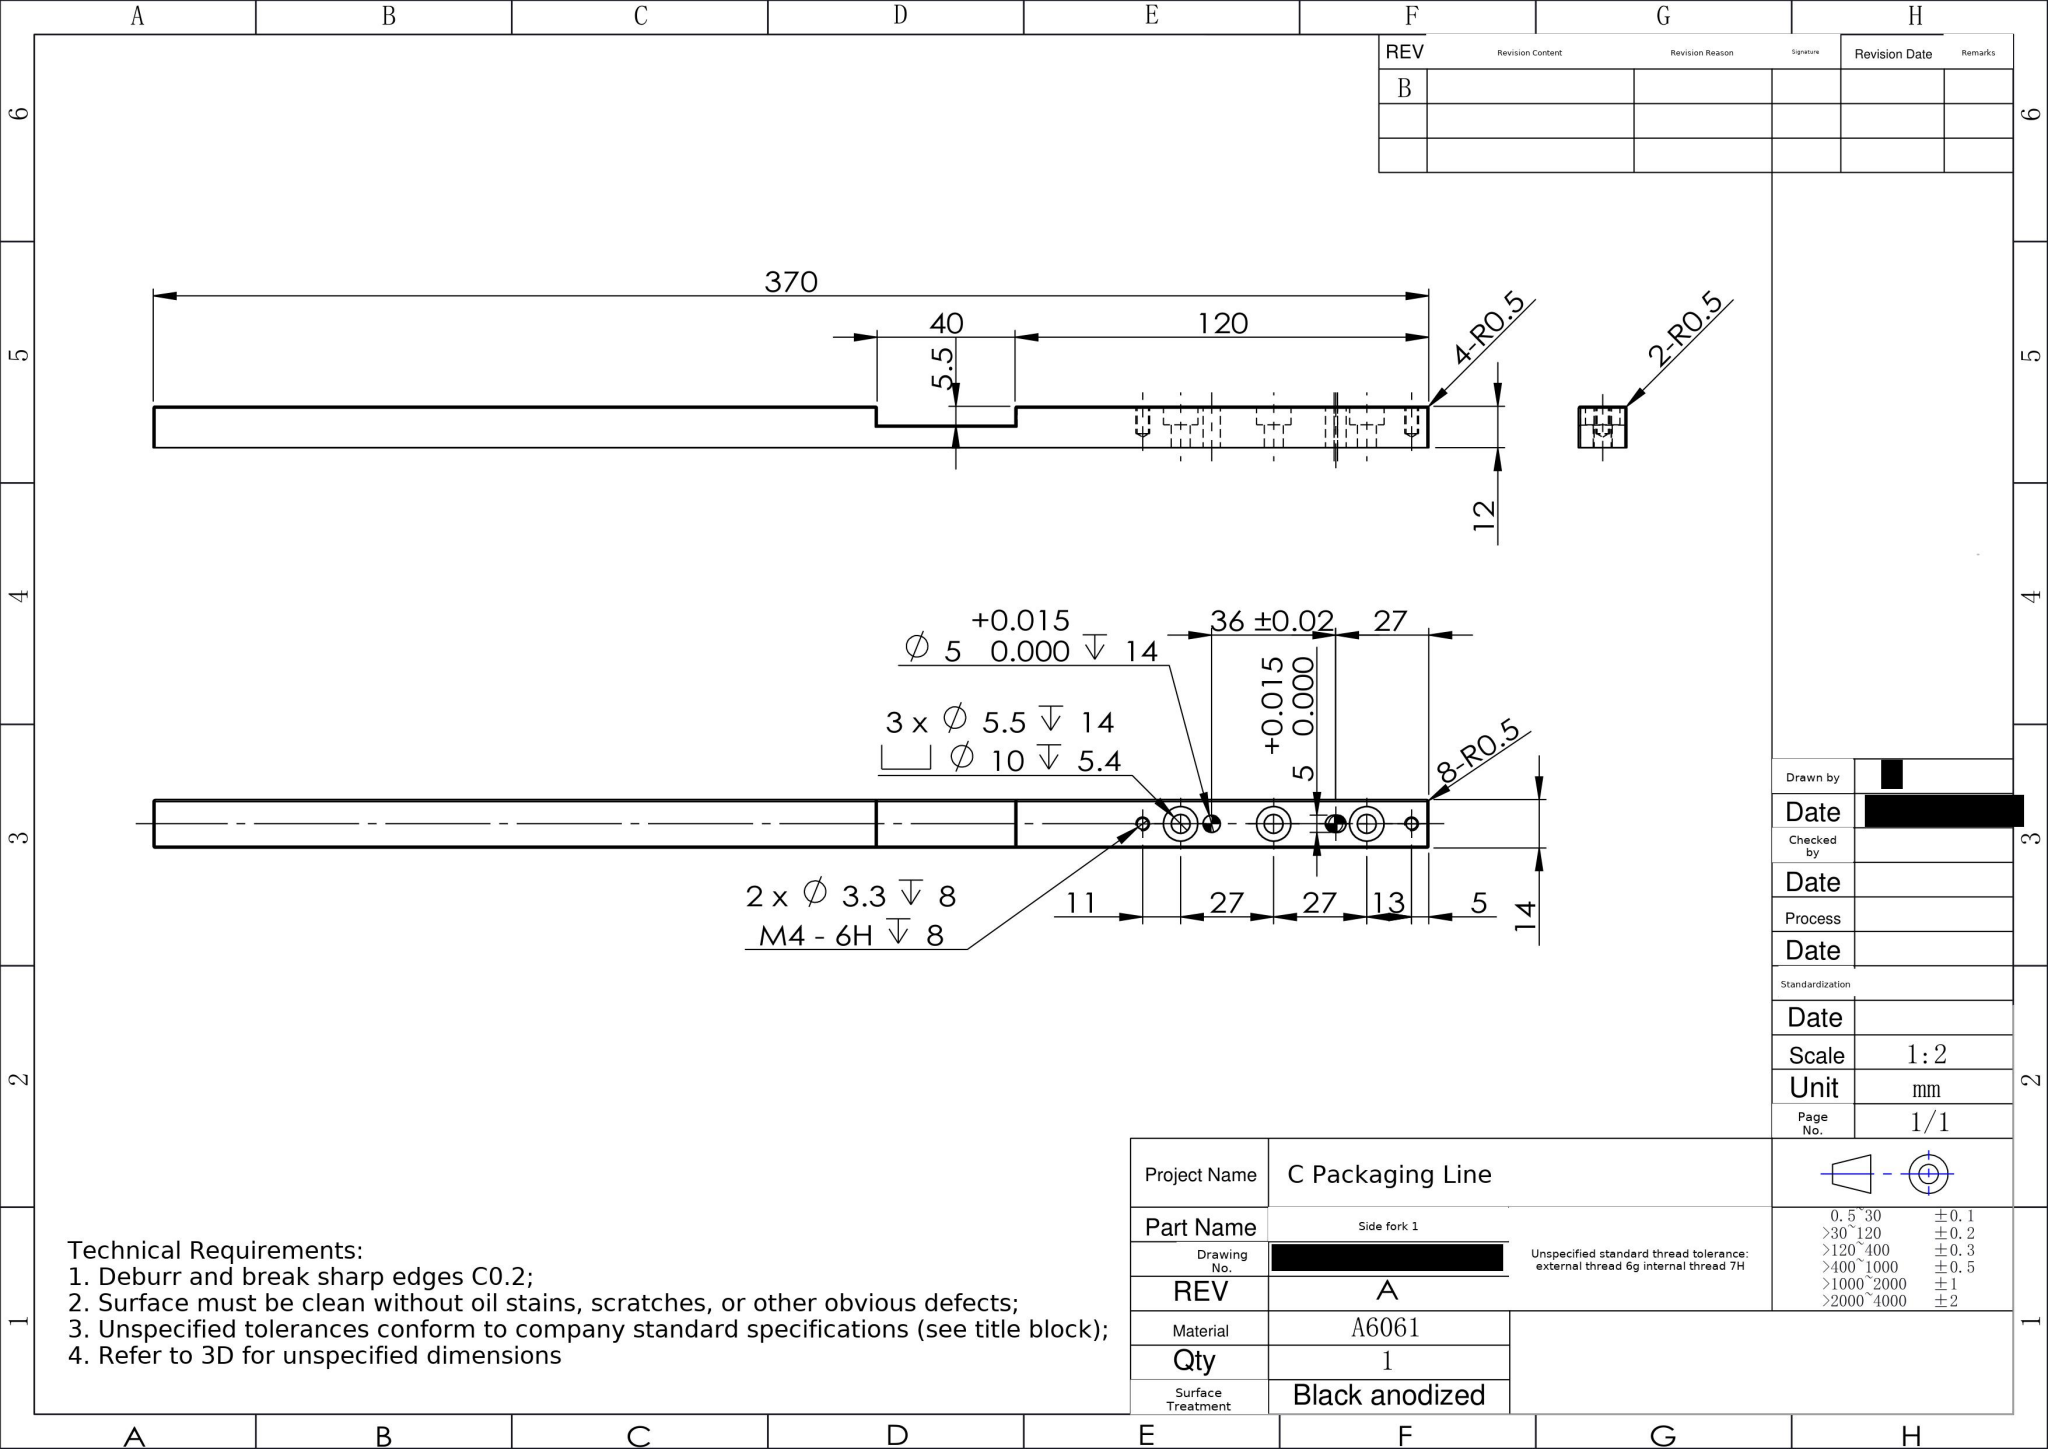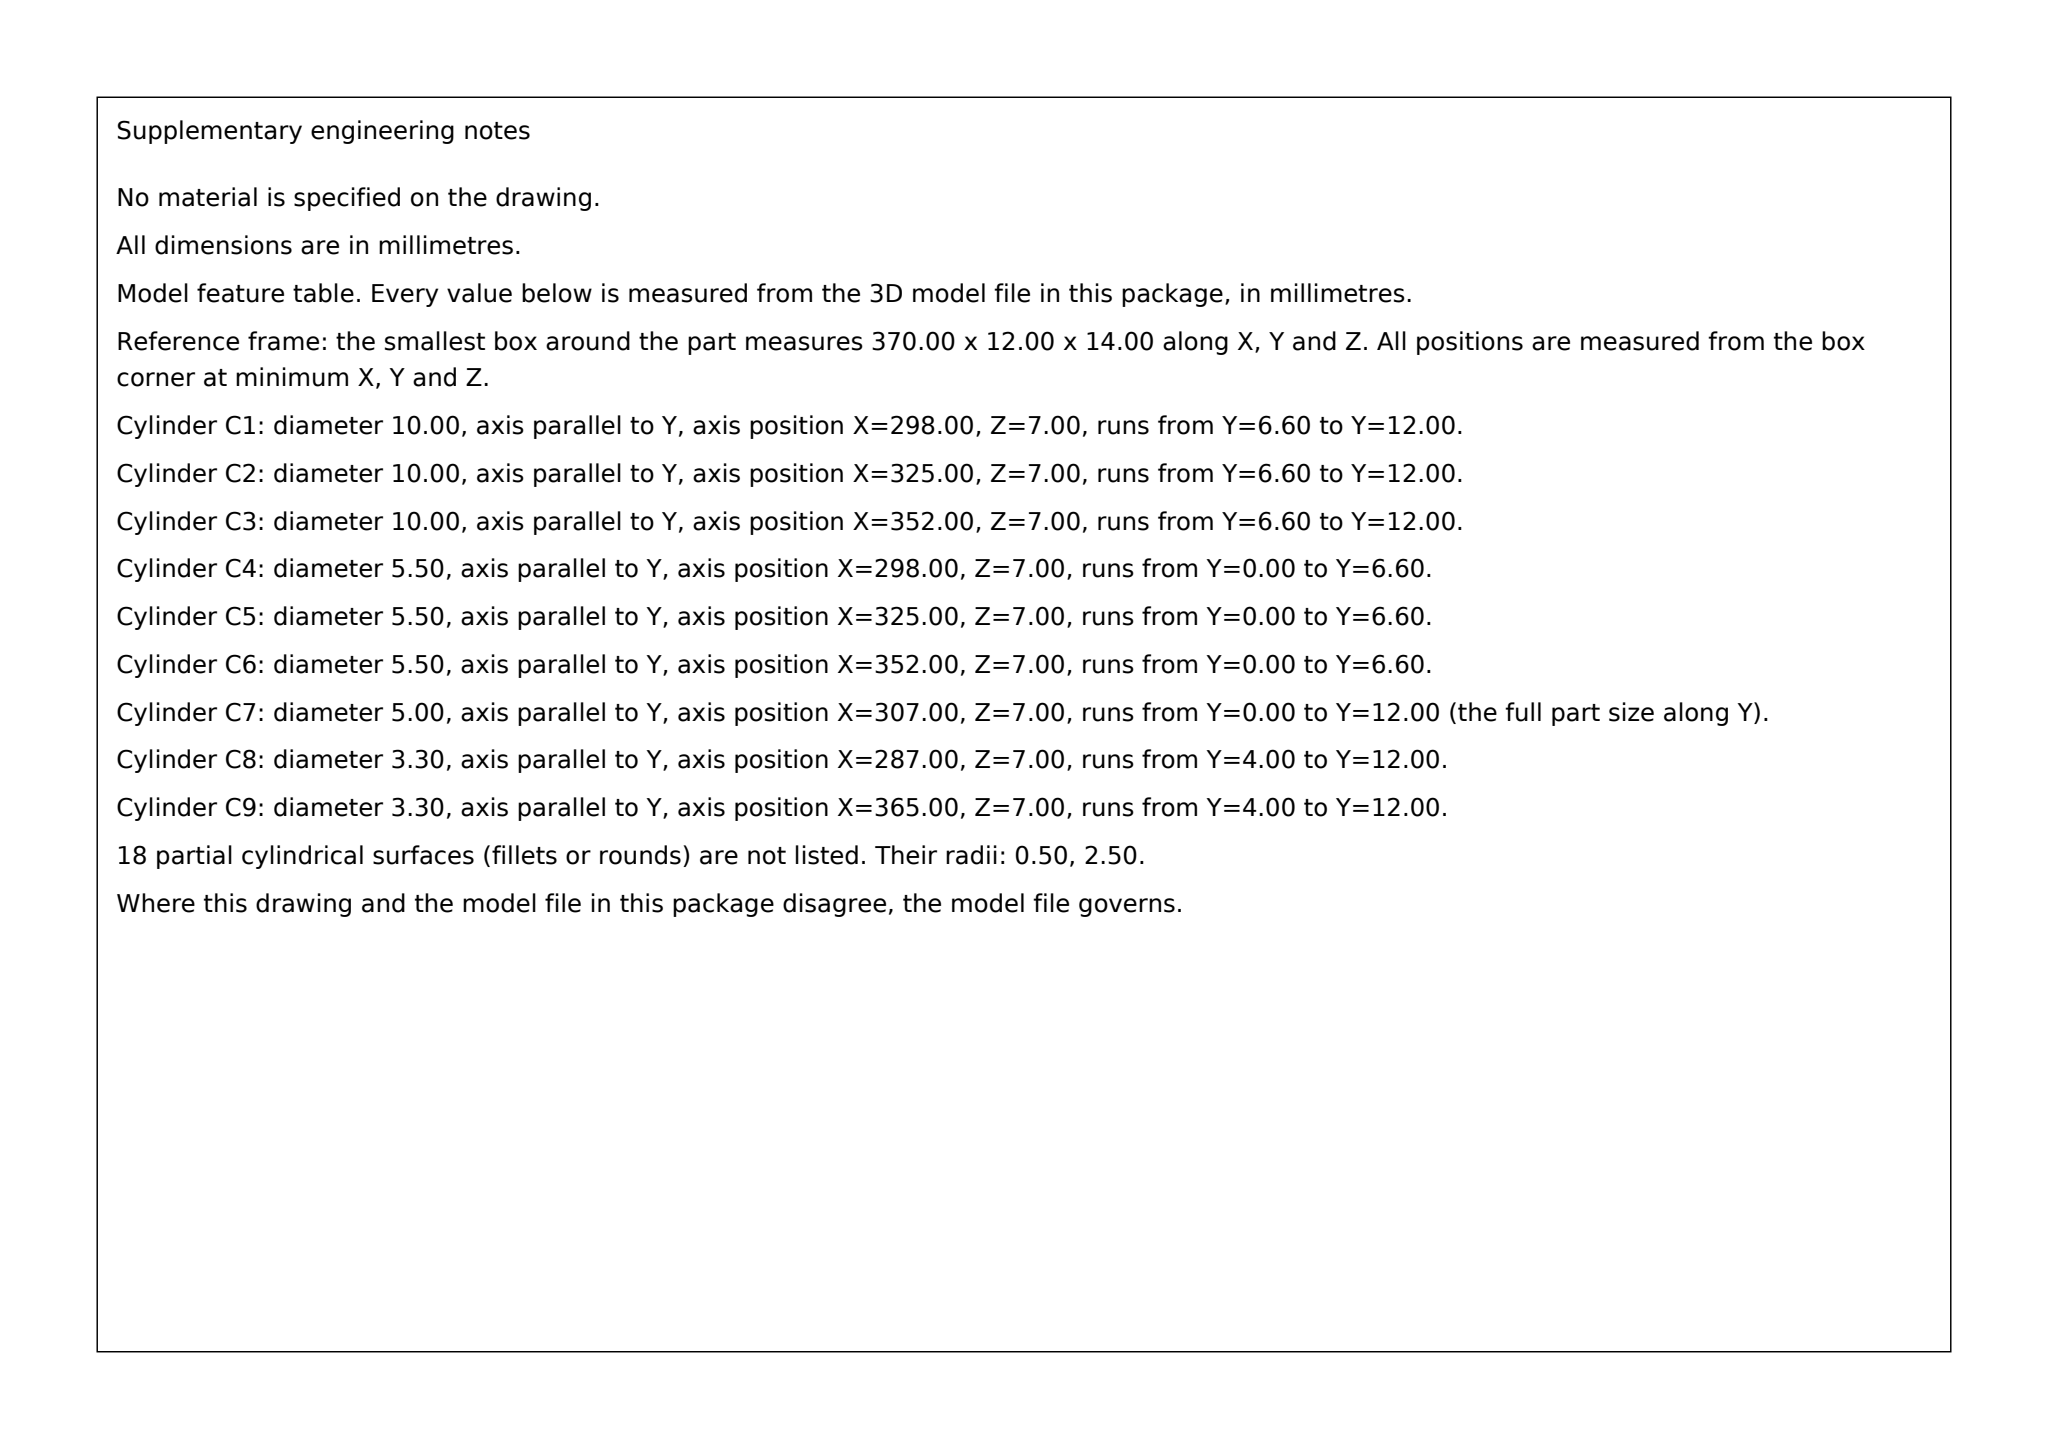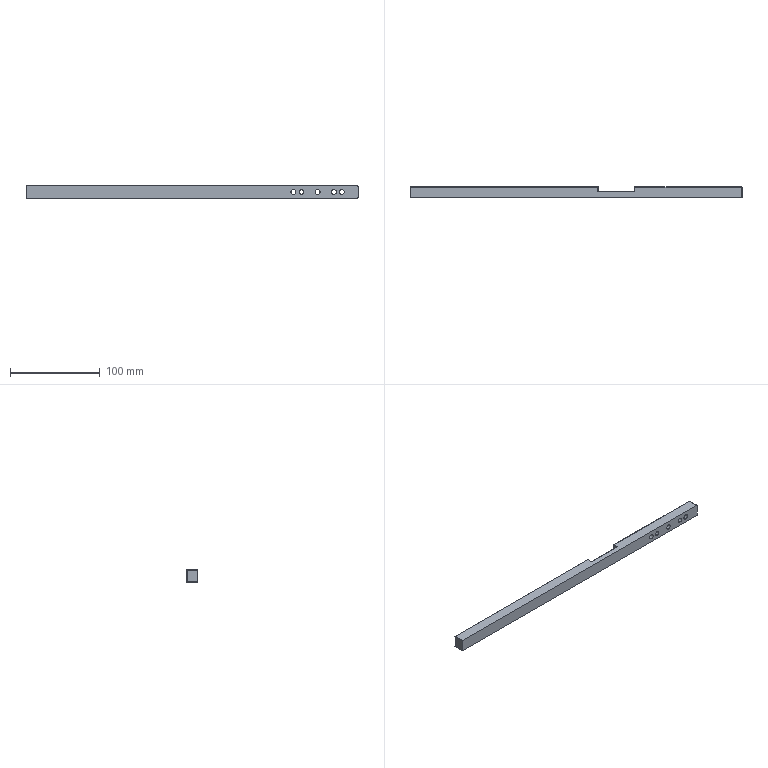Part | SolidWorks | mm | 1 solid | 65 faces | box 370 x 12 x 14 mm | volume 56617 mm3 | cylinder 38 | plane 15 | sphere 8 | cone 4 | commonest cylinder face diameters 1 x18 10 x6 5.5 x6 3.3 x4 5 x4